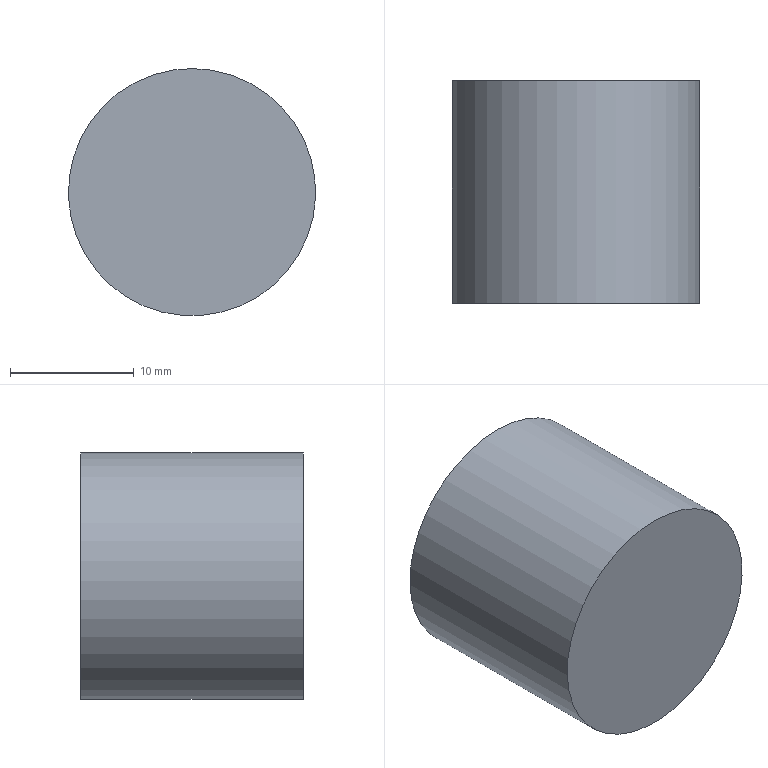Component | NX | MODEL5 | 1 solid | 3 faces | box 20 x 18 x 20 mm | volume 5655 mm3 | plane 2 | cylinder 1 | commonest cylinder face diameters 20 x1
STEP:
#1=CARTESIAN_POINT('',(0.,0.,0.));
#2=DIRECTION('',(0.,0.,1.));
#3=DIRECTION('',(1.,0.,0.));
#4=AXIS2_PLACEMENT_3D('',#1,#2,#3);
#5=CARTESIAN_POINT('',(7.918,-123.,45.204));
#6=VERTEX_POINT('',#5);
#7=CARTESIAN_POINT('',(16.603,-123.,50.161));
#8=DIRECTION('',(0.,1.,0.));
#9=DIRECTION('',(-0.8685,0.,-0.4957));
#10=AXIS2_PLACEMENT_3D('',#7,#8,#9);
#11=CIRCLE('',#10,10.);
#12=CARTESIAN_POINT('',(16.603,-123.,50.161));
#13=DIRECTION('',(0.,-1.,0.));
#14=DIRECTION('',(0.8685,0.,0.4957));
#15=AXIS2_PLACEMENT_3D('',#12,#13,#14);
#16=CYLINDRICAL_SURFACE('',#15,10.);
#17=CARTESIAN_POINT('',(9.425,0.));
#18=DIRECTION('',(-1.,0.));
#19=VECTOR('',#18,1.);
#20=LINE('',#17,#19);
#21=(GEOMETRIC_REPRESENTATION_CONTEXT(2)PARAMETRIC_REPRESENTATION_CONTEXT()REPRESENTATION_CONTEXT('',''));
#22=DEFINITIONAL_REPRESENTATION('',(#20),#21);
#23=PCURVE('',#16,#22);
#24=CARTESIAN_POINT('',(16.603,-123.,50.161));
#25=DIRECTION('',(0.,1.,0.));
#26=DIRECTION('',(-0.8685,0.,-0.4957));
#27=AXIS2_PLACEMENT_3D('',#24,#25,#26);
#28=PLANE('',#27);
#29=CARTESIAN_POINT('',(0.,0.));
#30=DIRECTION('',(1.,0.));
#31=AXIS2_PLACEMENT_2D('',#29,#30);
#32=CIRCLE('',#31,10.);
#33=(GEOMETRIC_REPRESENTATION_CONTEXT(2)PARAMETRIC_REPRESENTATION_CONTEXT()REPRESENTATION_CONTEXT('',''));
#34=DEFINITIONAL_REPRESENTATION('',(#32),#33);
#35=PCURVE('',#28,#34);
#36=SURFACE_CURVE('',#11,(#23,#35),.PCURVE_S1.);
#37=EDGE_CURVE('',#6,#6,#36,.T.);
#38=ORIENTED_EDGE('',*,*,#37,.F.);
#39=CARTESIAN_POINT('',(7.918,-141.,45.204));
#40=VERTEX_POINT('',#39);
#41=CARTESIAN_POINT('',(7.918,-123.,45.204));
#42=CARTESIAN_POINT('',(7.918,-141.,45.204));
#43=B_SPLINE_CURVE_WITH_KNOTS('',1,(#41,#42),.UNSPECIFIED.,.F.,.F.,(2,2),(0.,18.),.PIECEWISE_BEZIER_KNOTS.);
#44=CARTESIAN_POINT('',(9.425,0.));
#45=DIRECTION('',(0.,1.));
#46=VECTOR('',#45,1.);
#47=LINE('',#44,#46);
#48=(GEOMETRIC_REPRESENTATION_CONTEXT(2)PARAMETRIC_REPRESENTATION_CONTEXT()REPRESENTATION_CONTEXT('',''));
#49=DEFINITIONAL_REPRESENTATION('',(#47),#48);
#50=PCURVE('',#16,#49);
#51=CARTESIAN_POINT('',(3.142,0.));
#52=DIRECTION('',(0.,1.));
#53=VECTOR('',#52,1.);
#54=LINE('',#51,#53);
#55=(GEOMETRIC_REPRESENTATION_CONTEXT(2)PARAMETRIC_REPRESENTATION_CONTEXT()REPRESENTATION_CONTEXT('',''));
#56=DEFINITIONAL_REPRESENTATION('',(#54),#55);
#57=PCURVE('',#16,#56);
#58=SEAM_CURVE('',#43,(#50,#57),.PCURVE_S1.);
#59=EDGE_CURVE('',#6,#40,#58,.T.);
#60=ORIENTED_EDGE('',*,*,#59,.T.);
#61=CARTESIAN_POINT('',(16.603,-141.,50.161));
#62=DIRECTION('',(0.,1.,0.));
#63=DIRECTION('',(-0.8685,0.,-0.4957));
#64=AXIS2_PLACEMENT_3D('',#61,#62,#63);
#65=CIRCLE('',#64,10.);
#66=CARTESIAN_POINT('',(9.425,18.));
#67=DIRECTION('',(-1.,0.));
#68=VECTOR('',#67,1.);
#69=LINE('',#66,#68);
#70=(GEOMETRIC_REPRESENTATION_CONTEXT(2)PARAMETRIC_REPRESENTATION_CONTEXT()REPRESENTATION_CONTEXT('',''));
#71=DEFINITIONAL_REPRESENTATION('',(#69),#70);
#72=PCURVE('',#16,#71);
#73=CARTESIAN_POINT('',(16.603,-141.,50.161));
#74=DIRECTION('',(0.,1.,0.));
#75=DIRECTION('',(-0.8685,0.,-0.4957));
#76=AXIS2_PLACEMENT_3D('',#73,#74,#75);
#77=PLANE('',#76);
#78=CARTESIAN_POINT('',(0.,0.));
#79=DIRECTION('',(1.,0.));
#80=AXIS2_PLACEMENT_2D('',#78,#79);
#81=CIRCLE('',#80,10.);
#82=(GEOMETRIC_REPRESENTATION_CONTEXT(2)PARAMETRIC_REPRESENTATION_CONTEXT()REPRESENTATION_CONTEXT('',''));
#83=DEFINITIONAL_REPRESENTATION('',(#81),#82);
#84=PCURVE('',#77,#83);
#85=SURFACE_CURVE('',#65,(#72,#84),.PCURVE_S1.);
#86=EDGE_CURVE('',#40,#40,#85,.T.);
#87=ORIENTED_EDGE('',*,*,#86,.T.);
#88=ORIENTED_EDGE('',*,*,#59,.F.);
#89=EDGE_LOOP('',(#38,#60,#87,#88));
#90=FACE_BOUND('',#89,.T.);
#91=ADVANCED_FACE('',(#90),#16,.T.);
#92=ORIENTED_EDGE('',*,*,#37,.T.);
#93=EDGE_LOOP('',(#92));
#94=FACE_BOUND('',#93,.T.);
#95=ADVANCED_FACE('',(#94),#28,.T.);
#96=ORIENTED_EDGE('',*,*,#86,.F.);
#97=EDGE_LOOP('',(#96));
#98=FACE_BOUND('',#97,.T.);
#99=ADVANCED_FACE('',(#98),#77,.F.);
#100=CLOSED_SHELL('',(#91,#95,#99));
#101=MANIFOLD_SOLID_BREP('',#100);
#102=(LENGTH_UNIT()NAMED_UNIT(*)SI_UNIT(.MILLI.,.METRE.));
#103=UNCERTAINTY_MEASURE_WITH_UNIT(LENGTH_MEASURE(0.00001),#102,'','');
#104=(NAMED_UNIT(*)PLANE_ANGLE_UNIT()SI_UNIT($,.RADIAN.));
#105=(NAMED_UNIT(*)SI_UNIT($,.STERADIAN.)SOLID_ANGLE_UNIT());
#106=(GEOMETRIC_REPRESENTATION_CONTEXT(3)GLOBAL_UNCERTAINTY_ASSIGNED_CONTEXT((#103))GLOBAL_UNIT_ASSIGNED_CONTEXT((#102,#104,#105))REPRESENTATION_CONTEXT('',''));
#107=ADVANCED_BREP_SHAPE_REPRESENTATION('',(#4,#101),#106);